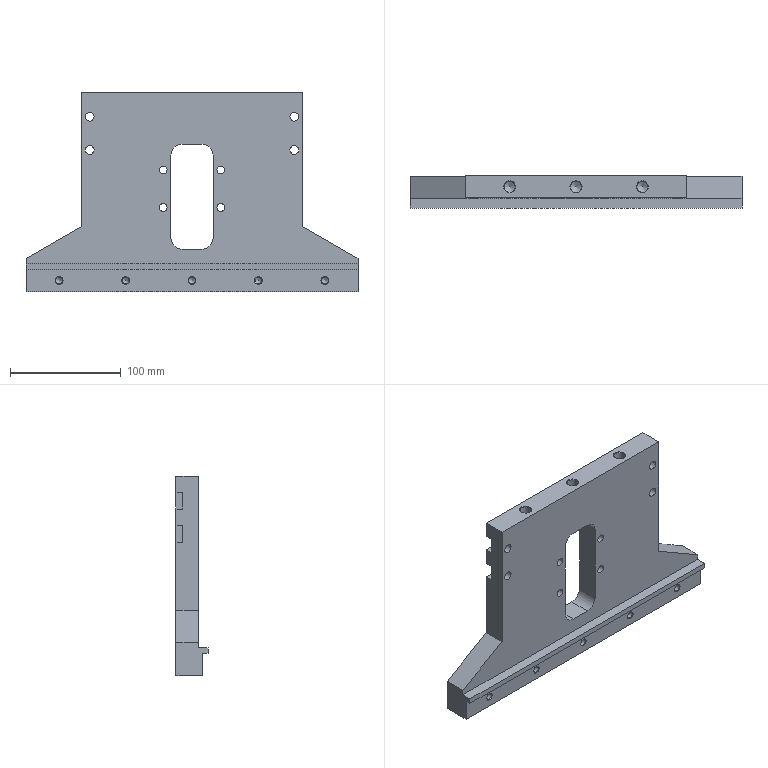Component | NX | CYL_FIX_VERT_PLATE | 1 solid | 78 faces | volume 752806 mm3 | plane 38 | cylinder 24 | cone 16 | commonest cylinder face diameters 6 x5 7 x4 8 x4 20 x4 12 x4 10 x3